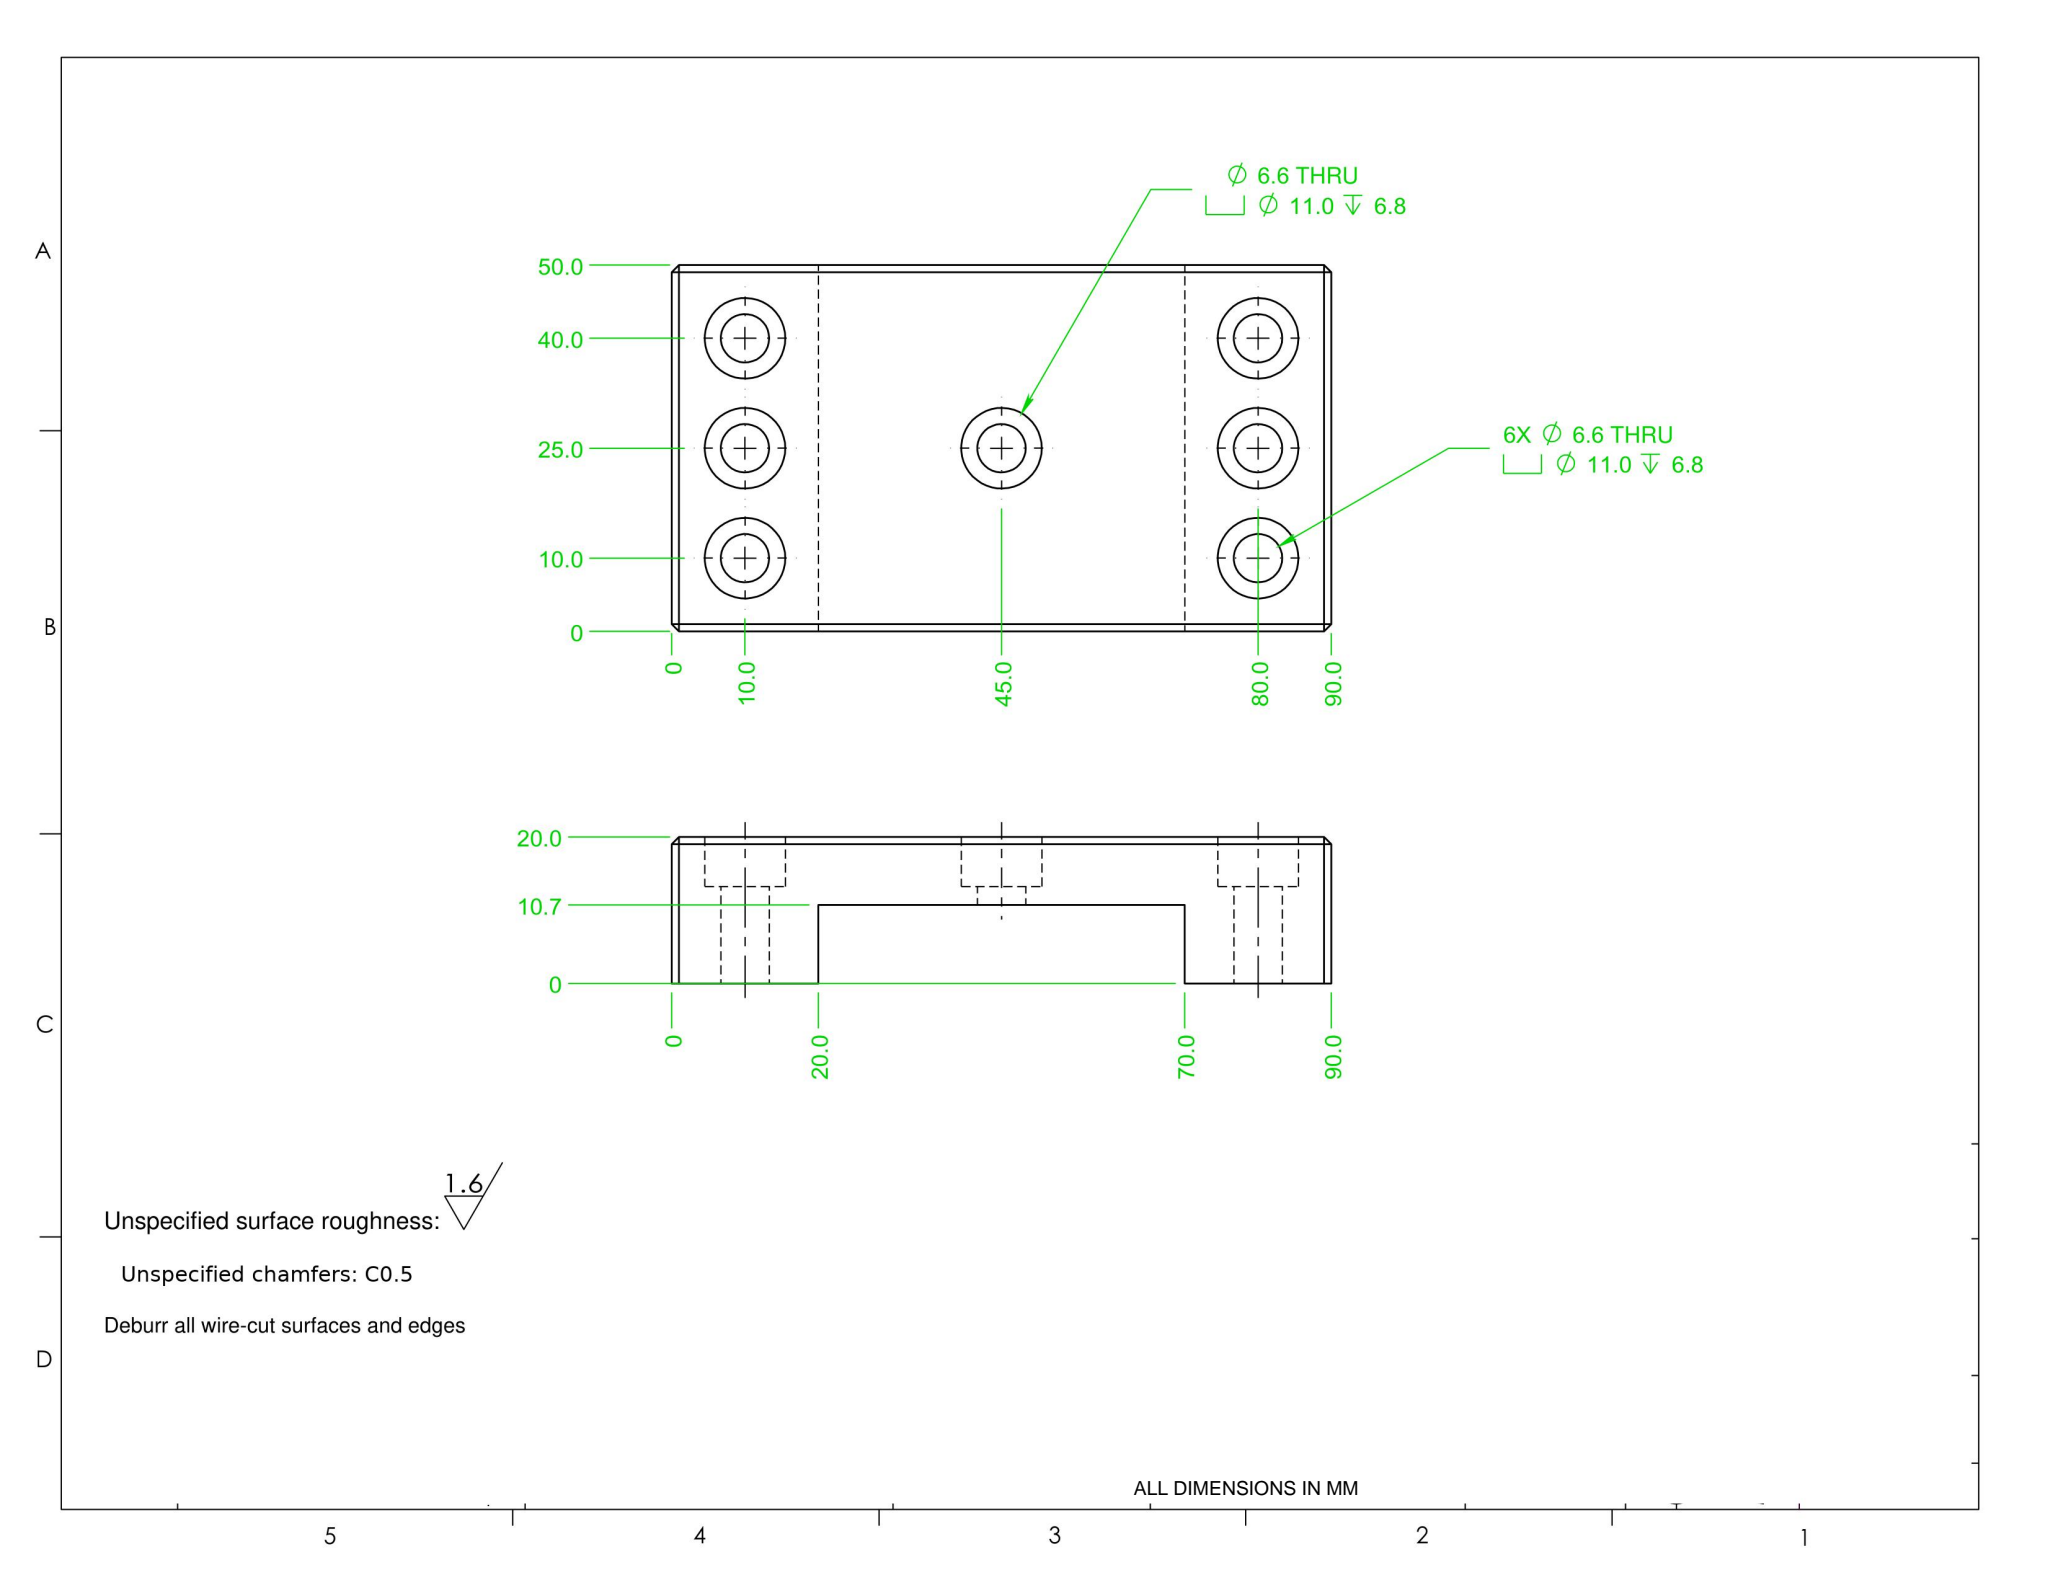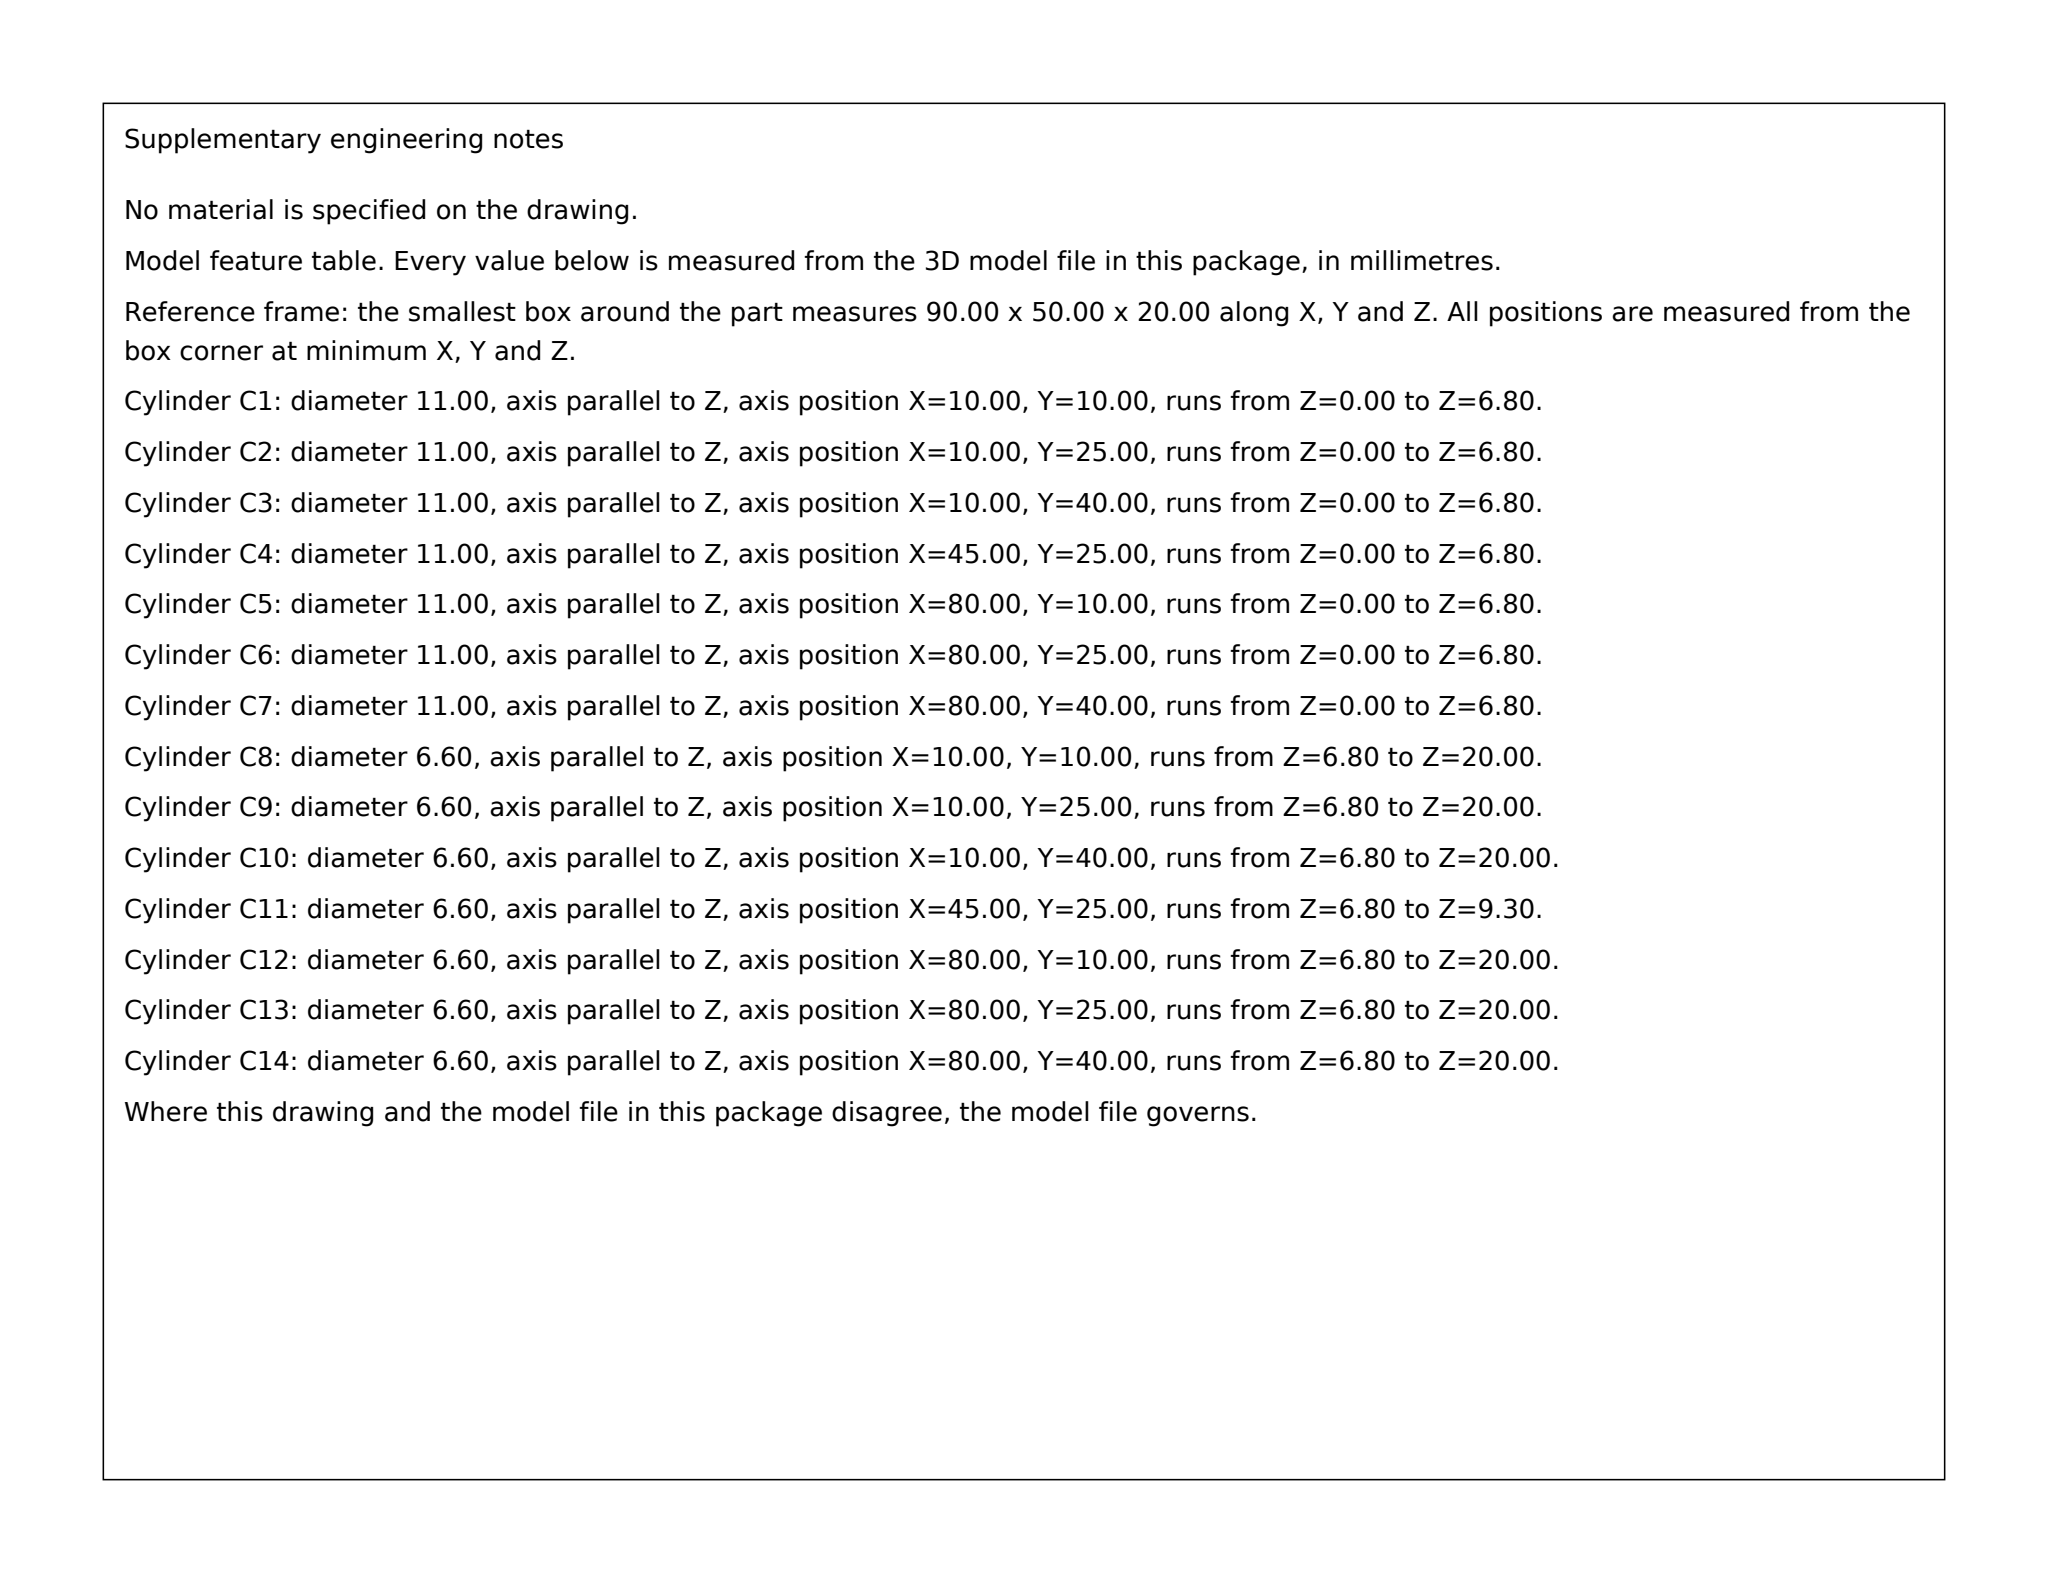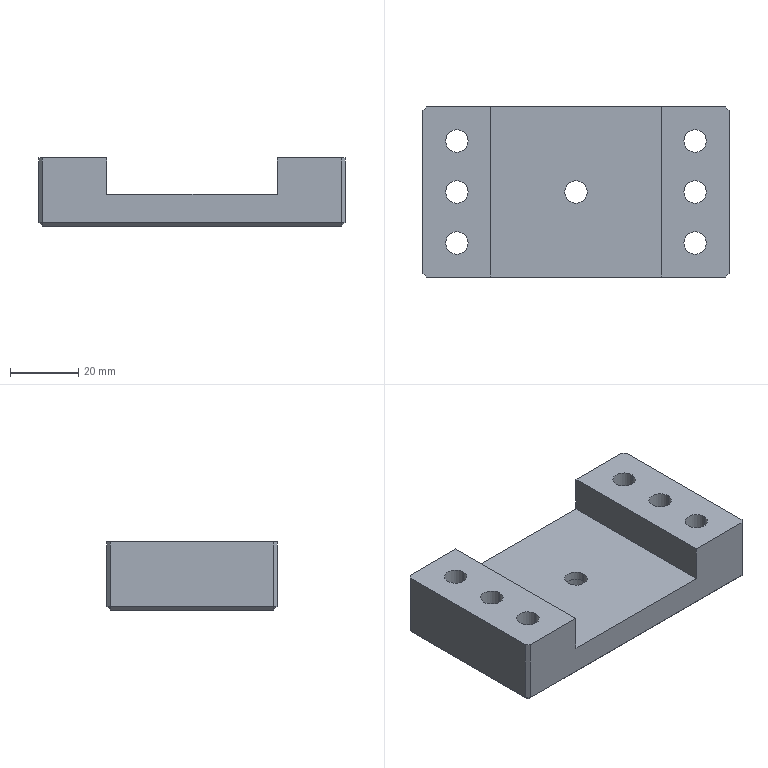Part | SolidWorks | mm | 1 solid | 57 faces | box 90 x 50 x 20 mm | volume 55754 mm3 | plane 29 | cylinder 28 | commonest cylinder face diameters 11 x14 6.6 x14
build123d program:
from build123d import *

# Parameters (mm, degrees)
SKETCH1_W                                         = 90
SKETCH1_H                                         = 50
BOSS_EXTRUDE1_DEPTH                               = 20
SKETCH2_W                                         = 50
SKETCH2_H                                         = 50
CUT_EXTRUDE1_DEPTH                                = 10.7
HOLE_SIZE_ACCORDING_TO_HEXAGON_SOCKET_D           = 6.6
HOLE_SIZE_ACCORDING_TO_HEXAGON_SOCKET_CBORE_D     = 11
HOLE_SIZE_ACCORDING_TO_HEXAGON_SOCKET_CBORE_DEPTH = 6.8
HOLE_SIZE_ACCORDING_TO_HEXAGON_SO_2_D             = 6.6
HOLE_SIZE_ACCORDING_TO_HEXAGON_SO_2_CBORE_D       = 11
HOLE_SIZE_ACCORDING_TO_HEXAGON_SO_2_CBORE_DEPTH   = 6.8
CHAMFER1_SIZE                                     = 1


with BuildPart() as part:
    # Sketch1 → Boss-Extrude1 (new body)
    with BuildSketch(Plane.XY):
        Rectangle(SKETCH1_W, SKETCH1_H)
    extrude(amount=BOSS_EXTRUDE1_DEPTH)

    # Sketch2 → Cut-Extrude1 (cut)
    with BuildSketch(Plane.XY.offset(20)):
        Rectangle(SKETCH2_W, SKETCH2_H)
    extrude(amount=-CUT_EXTRUDE1_DEPTH, mode=Mode.SUBTRACT)

    # Hole Size _ according to_ Hexagon Socket (through all)
    with Locations(Plane(origin=(0, 0, 0), x_dir=(-1, 0, 0), z_dir=(0, 0, -1))):
        with Locations((0, 0)):
            CounterBoreHole(HOLE_SIZE_ACCORDING_TO_HEXAGON_SOCKET_D / 2, HOLE_SIZE_ACCORDING_TO_HEXAGON_SOCKET_CBORE_D / 2, HOLE_SIZE_ACCORDING_TO_HEXAGON_SOCKET_CBORE_DEPTH)

    # Hole Size _ according to_ Hexagon So 2 (through all)
    with Locations(Plane(origin=(0, 0, 0), x_dir=(-1, 0, 0), z_dir=(0, 0, -1))):
        with Locations((35, 15), (35, 0), (35, -15), (-35, -15), (-35, 0), (-35, 15)):
            CounterBoreHole(HOLE_SIZE_ACCORDING_TO_HEXAGON_SO_2_D / 2, HOLE_SIZE_ACCORDING_TO_HEXAGON_SO_2_CBORE_D / 2, HOLE_SIZE_ACCORDING_TO_HEXAGON_SO_2_CBORE_DEPTH)

    # Chamfer1
    chamfer1_edges = [part.edges().sort_by_distance(p)[0] for p in [
        (0, 25, 0),
        (45, 0, 0),
        (0, -25, 0),
        (-45, 0, 0),
        (-45, 25, 10),
        (45, 25, 10),
        (45, -25, 10),
        (-45, -25, 10),
    ]]
    chamfer(chamfer1_edges, length=CHAMFER1_SIZE)


solid = part.part